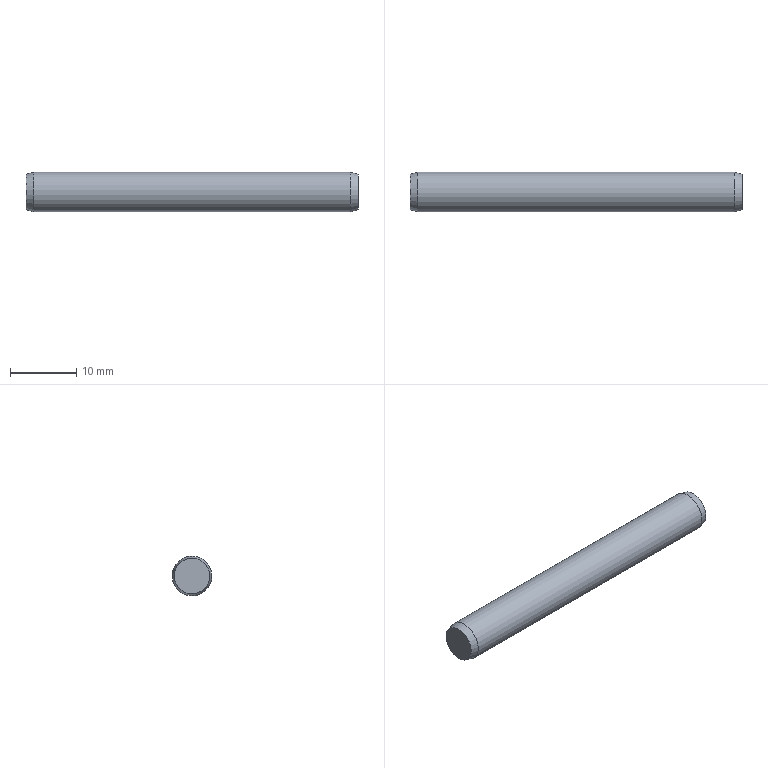Component | NX | GB-T119_1-2000_6X50 | 1 solid | 5 faces | box 50 x 6 x 6 mm | volume 1407 mm3 | plane 2 | cone 2 | cylinder 1 | commonest cylinder face diameters 6 x1
STEP:
#1=CARTESIAN_POINT('',(0.,0.,0.));
#2=DIRECTION('',(0.,0.,1.));
#3=DIRECTION('',(1.,0.,0.));
#4=AXIS2_PLACEMENT_3D('',#1,#2,#3);
#5=CARTESIAN_POINT('',(-40.,26.164,24.711));
#6=VERTEX_POINT('',#5);
#7=CARTESIAN_POINT('',(-40.,23.688,23.688));
#8=DIRECTION('',(-1.,0.,0.));
#9=DIRECTION('',(0.,0.9242,0.3818));
#10=AXIS2_PLACEMENT_3D('',#7,#8,#9);
#11=CIRCLE('',#10,2.678);
#12=CARTESIAN_POINT('',(-40.,23.688,23.688));
#13=DIRECTION('',(-1.,0.,0.));
#14=DIRECTION('',(0.,0.9242,0.3818));
#15=AXIS2_PLACEMENT_3D('',#12,#13,#14);
#16=PLANE('',#15);
#17=CARTESIAN_POINT('',(0.,-0.));
#18=DIRECTION('',(1.,0.));
#19=AXIS2_PLACEMENT_2D('',#17,#18);
#20=CIRCLE('',#19,2.678);
#21=(GEOMETRIC_REPRESENTATION_CONTEXT(2)PARAMETRIC_REPRESENTATION_CONTEXT()REPRESENTATION_CONTEXT('',''));
#22=DEFINITIONAL_REPRESENTATION('',(#20),#21);
#23=PCURVE('',#16,#22);
#24=CARTESIAN_POINT('',(-40.,23.688,23.688));
#25=DIRECTION('',(1.,0.,0.));
#26=DIRECTION('',(0.,-0.9242,-0.3818));
#27=AXIS2_PLACEMENT_3D('',#24,#25,#26);
#28=CONICAL_SURFACE('',#27,2.678,0.2618);
#29=CARTESIAN_POINT('',(9.425,0.));
#30=DIRECTION('',(-1.,0.));
#31=VECTOR('',#30,1.);
#32=LINE('',#29,#31);
#33=(GEOMETRIC_REPRESENTATION_CONTEXT(2)PARAMETRIC_REPRESENTATION_CONTEXT()REPRESENTATION_CONTEXT('',''));
#34=DEFINITIONAL_REPRESENTATION('',(#32),#33);
#35=PCURVE('',#28,#34);
#36=SURFACE_CURVE('',#11,(#23,#35),.PCURVE_S1.);
#37=EDGE_CURVE('',#6,#6,#36,.T.);
#38=ORIENTED_EDGE('',*,*,#37,.T.);
#39=EDGE_LOOP('',(#38));
#40=FACE_BOUND('',#39,.T.);
#41=ADVANCED_FACE('',(#40),#16,.T.);
#42=CARTESIAN_POINT('',(-38.8,26.461,24.834));
#43=VERTEX_POINT('',#42);
#44=CARTESIAN_POINT('',(-38.8,23.688,23.688));
#45=DIRECTION('',(-1.,0.,0.));
#46=DIRECTION('',(0.,0.9242,0.3818));
#47=AXIS2_PLACEMENT_3D('',#44,#45,#46);
#48=CIRCLE('',#47,3.);
#49=CARTESIAN_POINT('',(9.425,1.2));
#50=DIRECTION('',(-1.,0.));
#51=VECTOR('',#50,1.);
#52=LINE('',#49,#51);
#53=(GEOMETRIC_REPRESENTATION_CONTEXT(2)PARAMETRIC_REPRESENTATION_CONTEXT()REPRESENTATION_CONTEXT('',''));
#54=DEFINITIONAL_REPRESENTATION('',(#52),#53);
#55=PCURVE('',#28,#54);
#56=CARTESIAN_POINT('',(10.,23.688,23.688));
#57=DIRECTION('',(-1.,0.,0.));
#58=DIRECTION('',(0.,0.9242,0.3818));
#59=AXIS2_PLACEMENT_3D('',#56,#57,#58);
#60=CYLINDRICAL_SURFACE('',#59,3.);
#61=CARTESIAN_POINT('',(0.,48.8));
#62=DIRECTION('',(1.,0.));
#63=VECTOR('',#62,1.);
#64=LINE('',#61,#63);
#65=(GEOMETRIC_REPRESENTATION_CONTEXT(2)PARAMETRIC_REPRESENTATION_CONTEXT()REPRESENTATION_CONTEXT('',''));
#66=DEFINITIONAL_REPRESENTATION('',(#64),#65);
#67=PCURVE('',#60,#66);
#68=SURFACE_CURVE('',#48,(#55,#67),.PCURVE_S1.);
#69=EDGE_CURVE('',#43,#43,#68,.T.);
#70=ORIENTED_EDGE('',*,*,#69,.T.);
#71=CARTESIAN_POINT('',(-40.,26.164,24.711));
#72=CARTESIAN_POINT('',(-38.8,26.461,24.834));
#73=B_SPLINE_CURVE_WITH_KNOTS('',1,(#71,#72),.UNSPECIFIED.,.F.,.F.,(2,2),(0.,1.242),.PIECEWISE_BEZIER_KNOTS.);
#74=CARTESIAN_POINT('',(3.142,0.));
#75=DIRECTION('',(0.,1.));
#76=VECTOR('',#75,1.);
#77=LINE('',#74,#76);
#78=(GEOMETRIC_REPRESENTATION_CONTEXT(2)PARAMETRIC_REPRESENTATION_CONTEXT()REPRESENTATION_CONTEXT('',''));
#79=DEFINITIONAL_REPRESENTATION('',(#77),#78);
#80=PCURVE('',#28,#79);
#81=CARTESIAN_POINT('',(9.425,0.));
#82=DIRECTION('',(0.,1.));
#83=VECTOR('',#82,1.);
#84=LINE('',#81,#83);
#85=(GEOMETRIC_REPRESENTATION_CONTEXT(2)PARAMETRIC_REPRESENTATION_CONTEXT()REPRESENTATION_CONTEXT('',''));
#86=DEFINITIONAL_REPRESENTATION('',(#84),#85);
#87=PCURVE('',#28,#86);
#88=SEAM_CURVE('',#73,(#80,#87),.PCURVE_S1.);
#89=EDGE_CURVE('',#6,#43,#88,.T.);
#90=ORIENTED_EDGE('',*,*,#89,.F.);
#91=ORIENTED_EDGE('',*,*,#37,.F.);
#92=ORIENTED_EDGE('',*,*,#89,.T.);
#93=EDGE_LOOP('',(#70,#90,#91,#92));
#94=FACE_BOUND('',#93,.T.);
#95=ADVANCED_FACE('',(#94),#28,.T.);
#96=CARTESIAN_POINT('',(8.8,26.461,24.834));
#97=VERTEX_POINT('',#96);
#98=CARTESIAN_POINT('',(8.8,23.688,23.688));
#99=DIRECTION('',(-1.,0.,0.));
#100=DIRECTION('',(0.,0.9242,0.3818));
#101=AXIS2_PLACEMENT_3D('',#98,#99,#100);
#102=CIRCLE('',#101,3.);
#103=CARTESIAN_POINT('',(0.,1.2));
#104=DIRECTION('',(1.,0.));
#105=VECTOR('',#104,1.);
#106=LINE('',#103,#105);
#107=(GEOMETRIC_REPRESENTATION_CONTEXT(2)PARAMETRIC_REPRESENTATION_CONTEXT()REPRESENTATION_CONTEXT('',''));
#108=DEFINITIONAL_REPRESENTATION('',(#106),#107);
#109=PCURVE('',#60,#108);
#110=CARTESIAN_POINT('',(8.8,23.688,23.688));
#111=DIRECTION('',(-1.,0.,0.));
#112=DIRECTION('',(0.,0.9242,0.3818));
#113=AXIS2_PLACEMENT_3D('',#110,#111,#112);
#114=CONICAL_SURFACE('',#113,3.,0.2618);
#115=CARTESIAN_POINT('',(0.,0.));
#116=DIRECTION('',(1.,0.));
#117=VECTOR('',#116,1.);
#118=LINE('',#115,#117);
#119=(GEOMETRIC_REPRESENTATION_CONTEXT(2)PARAMETRIC_REPRESENTATION_CONTEXT()REPRESENTATION_CONTEXT('',''));
#120=DEFINITIONAL_REPRESENTATION('',(#118),#119);
#121=PCURVE('',#114,#120);
#122=SURFACE_CURVE('',#102,(#109,#121),.PCURVE_S1.);
#123=EDGE_CURVE('',#97,#97,#122,.T.);
#124=ORIENTED_EDGE('',*,*,#123,.T.);
#125=CARTESIAN_POINT('',(8.8,26.461,24.834));
#126=CARTESIAN_POINT('',(-38.8,26.461,24.834));
#127=B_SPLINE_CURVE_WITH_KNOTS('',1,(#125,#126),.UNSPECIFIED.,.F.,.F.,(2,2),(1.2,48.8),.PIECEWISE_BEZIER_KNOTS.);
#128=CARTESIAN_POINT('',(6.283,0.));
#129=DIRECTION('',(0.,1.));
#130=VECTOR('',#129,1.);
#131=LINE('',#128,#130);
#132=(GEOMETRIC_REPRESENTATION_CONTEXT(2)PARAMETRIC_REPRESENTATION_CONTEXT()REPRESENTATION_CONTEXT('',''));
#133=DEFINITIONAL_REPRESENTATION('',(#131),#132);
#134=PCURVE('',#60,#133);
#135=CARTESIAN_POINT('',(0.,0.));
#136=DIRECTION('',(0.,1.));
#137=VECTOR('',#136,1.);
#138=LINE('',#135,#137);
#139=(GEOMETRIC_REPRESENTATION_CONTEXT(2)PARAMETRIC_REPRESENTATION_CONTEXT()REPRESENTATION_CONTEXT('',''));
#140=DEFINITIONAL_REPRESENTATION('',(#138),#139);
#141=PCURVE('',#60,#140);
#142=SEAM_CURVE('',#127,(#134,#141),.PCURVE_S1.);
#143=EDGE_CURVE('',#97,#43,#142,.T.);
#144=ORIENTED_EDGE('',*,*,#143,.T.);
#145=ORIENTED_EDGE('',*,*,#69,.F.);
#146=ORIENTED_EDGE('',*,*,#143,.F.);
#147=EDGE_LOOP('',(#124,#144,#145,#146));
#148=FACE_BOUND('',#147,.T.);
#149=ADVANCED_FACE('',(#148),#60,.T.);
#150=CARTESIAN_POINT('',(10.,26.164,24.711));
#151=VERTEX_POINT('',#150);
#152=CARTESIAN_POINT('',(10.,23.688,23.688));
#153=DIRECTION('',(-1.,0.,0.));
#154=DIRECTION('',(0.,0.9242,0.3818));
#155=AXIS2_PLACEMENT_3D('',#152,#153,#154);
#156=CIRCLE('',#155,2.678);
#157=CARTESIAN_POINT('',(0.,-1.2));
#158=DIRECTION('',(1.,0.));
#159=VECTOR('',#158,1.);
#160=LINE('',#157,#159);
#161=(GEOMETRIC_REPRESENTATION_CONTEXT(2)PARAMETRIC_REPRESENTATION_CONTEXT()REPRESENTATION_CONTEXT('',''));
#162=DEFINITIONAL_REPRESENTATION('',(#160),#161);
#163=PCURVE('',#114,#162);
#164=CARTESIAN_POINT('',(10.,21.213,22.665));
#165=DIRECTION('',(1.,0.,0.));
#166=DIRECTION('',(0.,-0.9242,-0.3818));
#167=AXIS2_PLACEMENT_3D('',#164,#165,#166);
#168=PLANE('',#167);
#169=CARTESIAN_POINT('',(-5.357,-0.));
#170=CARTESIAN_POINT('',(-5.357,4.639));
#171=CARTESIAN_POINT('',(-1.339,2.32));
#172=CARTESIAN_POINT('',(2.678,-0.));
#173=CARTESIAN_POINT('',(-1.339,-2.32));
#174=CARTESIAN_POINT('',(-5.357,-4.639));
#175=CARTESIAN_POINT('',(-5.357,-0.));
#176=(BOUNDED_CURVE()B_SPLINE_CURVE(2,(#169,#170,#171,#172,#173,#174,#175),.UNSPECIFIED.,.T.,.F.)B_SPLINE_CURVE_WITH_KNOTS((1,2,2,2,2,1),(-2.094,0.,2.094,4.189,6.283,8.378),.UNSPECIFIED.)CURVE()GEOMETRIC_REPRESENTATION_ITEM()RATIONAL_B_SPLINE_CURVE((1.,0.5,1.,0.5,1.,0.5,1.))REPRESENTATION_ITEM(''));
#177=(GEOMETRIC_REPRESENTATION_CONTEXT(2)PARAMETRIC_REPRESENTATION_CONTEXT()REPRESENTATION_CONTEXT('',''));
#178=DEFINITIONAL_REPRESENTATION('',(#176),#177);
#179=PCURVE('',#168,#178);
#180=SURFACE_CURVE('',#156,(#163,#179),.PCURVE_S1.);
#181=EDGE_CURVE('',#151,#151,#180,.T.);
#182=ORIENTED_EDGE('',*,*,#181,.T.);
#183=CARTESIAN_POINT('',(10.,26.164,24.711));
#184=CARTESIAN_POINT('',(8.8,26.461,24.834));
#185=B_SPLINE_CURVE_WITH_KNOTS('',1,(#183,#184),.UNSPECIFIED.,.F.,.F.,(2,2),(-1.242,0.),.PIECEWISE_BEZIER_KNOTS.);
#186=CARTESIAN_POINT('',(6.283,0.));
#187=DIRECTION('',(0.,1.));
#188=VECTOR('',#187,1.);
#189=LINE('',#186,#188);
#190=(GEOMETRIC_REPRESENTATION_CONTEXT(2)PARAMETRIC_REPRESENTATION_CONTEXT()REPRESENTATION_CONTEXT('',''));
#191=DEFINITIONAL_REPRESENTATION('',(#189),#190);
#192=PCURVE('',#114,#191);
#193=CARTESIAN_POINT('',(0.,0.));
#194=DIRECTION('',(0.,1.));
#195=VECTOR('',#194,1.);
#196=LINE('',#193,#195);
#197=(GEOMETRIC_REPRESENTATION_CONTEXT(2)PARAMETRIC_REPRESENTATION_CONTEXT()REPRESENTATION_CONTEXT('',''));
#198=DEFINITIONAL_REPRESENTATION('',(#196),#197);
#199=PCURVE('',#114,#198);
#200=SEAM_CURVE('',#185,(#192,#199),.PCURVE_S1.);
#201=EDGE_CURVE('',#151,#97,#200,.T.);
#202=ORIENTED_EDGE('',*,*,#201,.T.);
#203=ORIENTED_EDGE('',*,*,#123,.F.);
#204=ORIENTED_EDGE('',*,*,#201,.F.);
#205=EDGE_LOOP('',(#182,#202,#203,#204));
#206=FACE_BOUND('',#205,.T.);
#207=ADVANCED_FACE('',(#206),#114,.T.);
#208=ORIENTED_EDGE('',*,*,#181,.F.);
#209=EDGE_LOOP('',(#208));
#210=FACE_BOUND('',#209,.T.);
#211=ADVANCED_FACE('',(#210),#168,.T.);
#212=CLOSED_SHELL('',(#41,#95,#149,#207,#211));
#213=MANIFOLD_SOLID_BREP('',#212);
#214=(LENGTH_UNIT()NAMED_UNIT(*)SI_UNIT(.MILLI.,.METRE.));
#215=UNCERTAINTY_MEASURE_WITH_UNIT(LENGTH_MEASURE(0.00001),#214,'','');
#216=(NAMED_UNIT(*)PLANE_ANGLE_UNIT()SI_UNIT($,.RADIAN.));
#217=(NAMED_UNIT(*)SI_UNIT($,.STERADIAN.)SOLID_ANGLE_UNIT());
#218=(GEOMETRIC_REPRESENTATION_CONTEXT(3)GLOBAL_UNCERTAINTY_ASSIGNED_CONTEXT((#215))GLOBAL_UNIT_ASSIGNED_CONTEXT((#214,#216,#217))REPRESENTATION_CONTEXT('',''));
#219=ADVANCED_BREP_SHAPE_REPRESENTATION('',(#4,#213),#218);